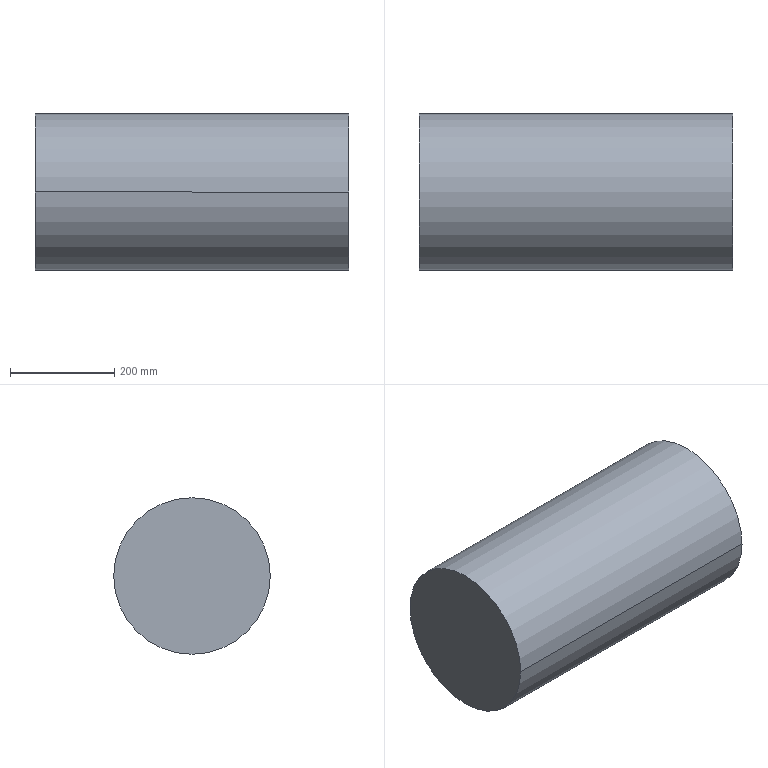Component | SolidWorks | LiftingAndOperatingMechanism-1_Part17-1 | 1 solid | 4 faces | box 600 x 300 x 300 mm | volume 42411501 mm3 | cylinder 2 | plane 2 | commonest cylinder face diameters 300 x2
build123d program:
from build123d import *

# Parameters (mm, degrees)
SKETCH1_R           = 150
BOSS_EXTRUDE1_DEPTH = 300


with BuildPart() as part:
    # Sketch1 → Boss-Extrude1 (new, symmetric)
    with BuildSketch(Plane(origin=(0, 0, 0), x_dir=(1, 0, 0), z_dir=(0, 1, 0))):
        with Locations(Location((0, 0, 0), (0, 0, 270))):
            Circle(SKETCH1_R)
    extrude(amount=BOSS_EXTRUDE1_DEPTH, both=True)


solid = part.part

# Placed as in the assembly
solid = solid.moved(Location((2876.037, 13568.918, 4082.152), (0, 0, 90)))
STEP:
#1=CARTESIAN_POINT('',(101.419,540.115,160.715));
#2=VERTEX_POINT('',#1);
#3=CARTESIAN_POINT('',(101.419,528.304,160.715));
#4=VERTEX_POINT('',#3);
#5=CARTESIAN_POINT('',(101.419,534.209,160.715));
#6=DIRECTION('',(-1.,-0.,0.0000002));
#7=DIRECTION('',(0.,1.,0.));
#8=AXIS2_PLACEMENT_3D('',#5,#6,#7);
#9=CIRCLE('',#8,5.906);
#10=EDGE_CURVE('',#2,#4,#9,.T.);
#11=ORIENTED_EDGE('',*,*,#10,.F.);
#12=CARTESIAN_POINT('',(125.041,540.115,160.715));
#13=VERTEX_POINT('',#12);
#14=CARTESIAN_POINT('',(101.419,540.115,160.715));
#15=DIRECTION('',(1.,0.,-0.0000002));
#16=VECTOR('',#15,39.37);
#17=LINE('',#14,#16);
#18=EDGE_CURVE('',#2,#13,#17,.T.);
#19=ORIENTED_EDGE('',*,*,#18,.T.);
#20=CARTESIAN_POINT('',(125.041,528.304,160.715));
#21=VERTEX_POINT('',#20);
#22=CARTESIAN_POINT('',(125.041,534.209,160.715));
#23=DIRECTION('',(-1.,-0.,0.0000002));
#24=DIRECTION('',(0.,1.,0.));
#25=AXIS2_PLACEMENT_3D('',#22,#23,#24);
#26=CIRCLE('',#25,5.906);
#27=EDGE_CURVE('',#13,#21,#26,.T.);
#28=ORIENTED_EDGE('',*,*,#27,.T.);
#29=CARTESIAN_POINT('',(101.419,528.304,160.715));
#30=DIRECTION('',(1.,0.,-0.0000002));
#31=VECTOR('',#30,39.37);
#32=LINE('',#29,#31);
#33=EDGE_CURVE('',#4,#21,#32,.T.);
#34=ORIENTED_EDGE('',*,*,#33,.F.);
#35=EDGE_LOOP('',(#11,#19,#28,#34));
#36=FACE_OUTER_BOUND('',#35,.T.);
#37=CARTESIAN_POINT('',(101.419,534.209,160.715));
#38=DIRECTION('',(1.,0.,-0.0000002));
#39=DIRECTION('',(0.,-1.,0.));
#40=AXIS2_PLACEMENT_3D('',#37,#38,#39);
#41=CYLINDRICAL_SURFACE('',#40,5.906);
#42=ADVANCED_FACE('',(#36),#41,.T.);
#43=ORIENTED_EDGE('',*,*,#18,.F.);
#44=CARTESIAN_POINT('',(101.419,534.209,160.715));
#45=DIRECTION('',(-1.,-0.,0.0000002));
#46=DIRECTION('',(0.,1.,0.));
#47=AXIS2_PLACEMENT_3D('',#44,#45,#46);
#48=CIRCLE('',#47,5.906);
#49=EDGE_CURVE('',#4,#2,#48,.T.);
#50=ORIENTED_EDGE('',*,*,#49,.F.);
#51=ORIENTED_EDGE('',*,*,#33,.T.);
#52=CARTESIAN_POINT('',(125.041,534.209,160.715));
#53=DIRECTION('',(-1.,-0.,0.0000002));
#54=DIRECTION('',(0.,1.,0.));
#55=AXIS2_PLACEMENT_3D('',#52,#53,#54);
#56=CIRCLE('',#55,5.906);
#57=EDGE_CURVE('',#21,#13,#56,.T.);
#58=ORIENTED_EDGE('',*,*,#57,.T.);
#59=EDGE_LOOP('',(#43,#50,#51,#58));
#60=FACE_OUTER_BOUND('',#59,.T.);
#61=CARTESIAN_POINT('',(101.419,534.209,160.715));
#62=DIRECTION('',(1.,0.,-0.0000002));
#63=DIRECTION('',(0.,-1.,0.));
#64=AXIS2_PLACEMENT_3D('',#61,#62,#63);
#65=CYLINDRICAL_SURFACE('',#64,5.906);
#66=ADVANCED_FACE('',(#60),#65,.T.);
#67=ORIENTED_EDGE('',*,*,#49,.T.);
#68=ORIENTED_EDGE('',*,*,#10,.T.);
#69=EDGE_LOOP('',(#67,#68));
#70=FACE_OUTER_BOUND('',#69,.T.);
#71=CARTESIAN_POINT('',(101.419,534.209,160.715));
#72=DIRECTION('',(-1.,-0.,0.0000002));
#73=DIRECTION('',(-0.,1.,0.));
#74=AXIS2_PLACEMENT_3D('',#71,#72,#73);
#75=PLANE('',#74);
#76=ADVANCED_FACE('',(#70),#75,.T.);
#77=ORIENTED_EDGE('',*,*,#57,.F.);
#78=ORIENTED_EDGE('',*,*,#27,.F.);
#79=EDGE_LOOP('',(#77,#78));
#80=FACE_OUTER_BOUND('',#79,.T.);
#81=CARTESIAN_POINT('',(125.041,534.209,160.715));
#82=DIRECTION('',(-1.,-0.,0.0000002));
#83=DIRECTION('',(-0.,1.,0.));
#84=AXIS2_PLACEMENT_3D('',#81,#82,#83);
#85=PLANE('',#84);
#86=ADVANCED_FACE('',(#80),#85,.F.);
#87=CLOSED_SHELL('',(#42,#66,#76,#86));
#88=MANIFOLD_SOLID_BREP('',#87);
#89=CARTESIAN_POINT('',(0.,0.,0.));
#90=DIRECTION('',(0.,0.,1.));
#91=DIRECTION('',(1.,0.,0.));
#92=AXIS2_PLACEMENT_3D('',#89,#90,#91);
#93=(LENGTH_UNIT()NAMED_UNIT(*)SI_UNIT($,.METRE.));
#94=LENGTH_MEASURE_WITH_UNIT(LENGTH_MEASURE(0.0254),#93);
#95=DIMENSIONAL_EXPONENTS(1.,0.,0.,0.,0.,0.,0.);
#96=(CONVERSION_BASED_UNIT('',#94)LENGTH_UNIT()NAMED_UNIT(#95));
#97=UNCERTAINTY_MEASURE_WITH_UNIT(LENGTH_MEASURE(0.00001),#96,'','');
#98=(NAMED_UNIT(*)PLANE_ANGLE_UNIT()SI_UNIT($,.RADIAN.));
#99=(NAMED_UNIT(*)SI_UNIT($,.STERADIAN.)SOLID_ANGLE_UNIT());
#100=(GEOMETRIC_REPRESENTATION_CONTEXT(3)GLOBAL_UNCERTAINTY_ASSIGNED_CONTEXT((#97))GLOBAL_UNIT_ASSIGNED_CONTEXT((#96,#98,#99))REPRESENTATION_CONTEXT('',''));
#101=ADVANCED_BREP_SHAPE_REPRESENTATION('',(#88,#92),#100);
#102=COLOUR_RGB('',0.7922,0.8196,0.9333);
#103=FILL_AREA_STYLE_COLOUR('',#102);
#104=FILL_AREA_STYLE('',(#103));
#105=SURFACE_STYLE_FILL_AREA(#104);
#106=SURFACE_SIDE_STYLE('',(#105));
#107=SURFACE_STYLE_USAGE(.BOTH.,#106);
#108=PRESENTATION_STYLE_ASSIGNMENT((#107));
#109=STYLED_ITEM('',(#108),#88);
#110=PRESENTATION_LAYER_ASSIGNMENT('','',(#109));
#111=(LENGTH_UNIT()NAMED_UNIT(*)SI_UNIT($,.METRE.));
#112=LENGTH_MEASURE_WITH_UNIT(LENGTH_MEASURE(0.0254),#111);
#113=DIMENSIONAL_EXPONENTS(1.,0.,0.,0.,0.,0.,0.);
#114=(CONVERSION_BASED_UNIT('',#112)LENGTH_UNIT()NAMED_UNIT(#113));
#115=UNCERTAINTY_MEASURE_WITH_UNIT(LENGTH_MEASURE(0.00001),#114,'','');
#116=(NAMED_UNIT(*)PLANE_ANGLE_UNIT()SI_UNIT($,.RADIAN.));
#117=(NAMED_UNIT(*)SI_UNIT($,.STERADIAN.)SOLID_ANGLE_UNIT());
#118=(GEOMETRIC_REPRESENTATION_CONTEXT(3)GLOBAL_UNCERTAINTY_ASSIGNED_CONTEXT((#115))GLOBAL_UNIT_ASSIGNED_CONTEXT((#114,#116,#117))REPRESENTATION_CONTEXT('',''));
#119=MECHANICAL_DESIGN_GEOMETRIC_PRESENTATION_REPRESENTATION('',(#109),#118);